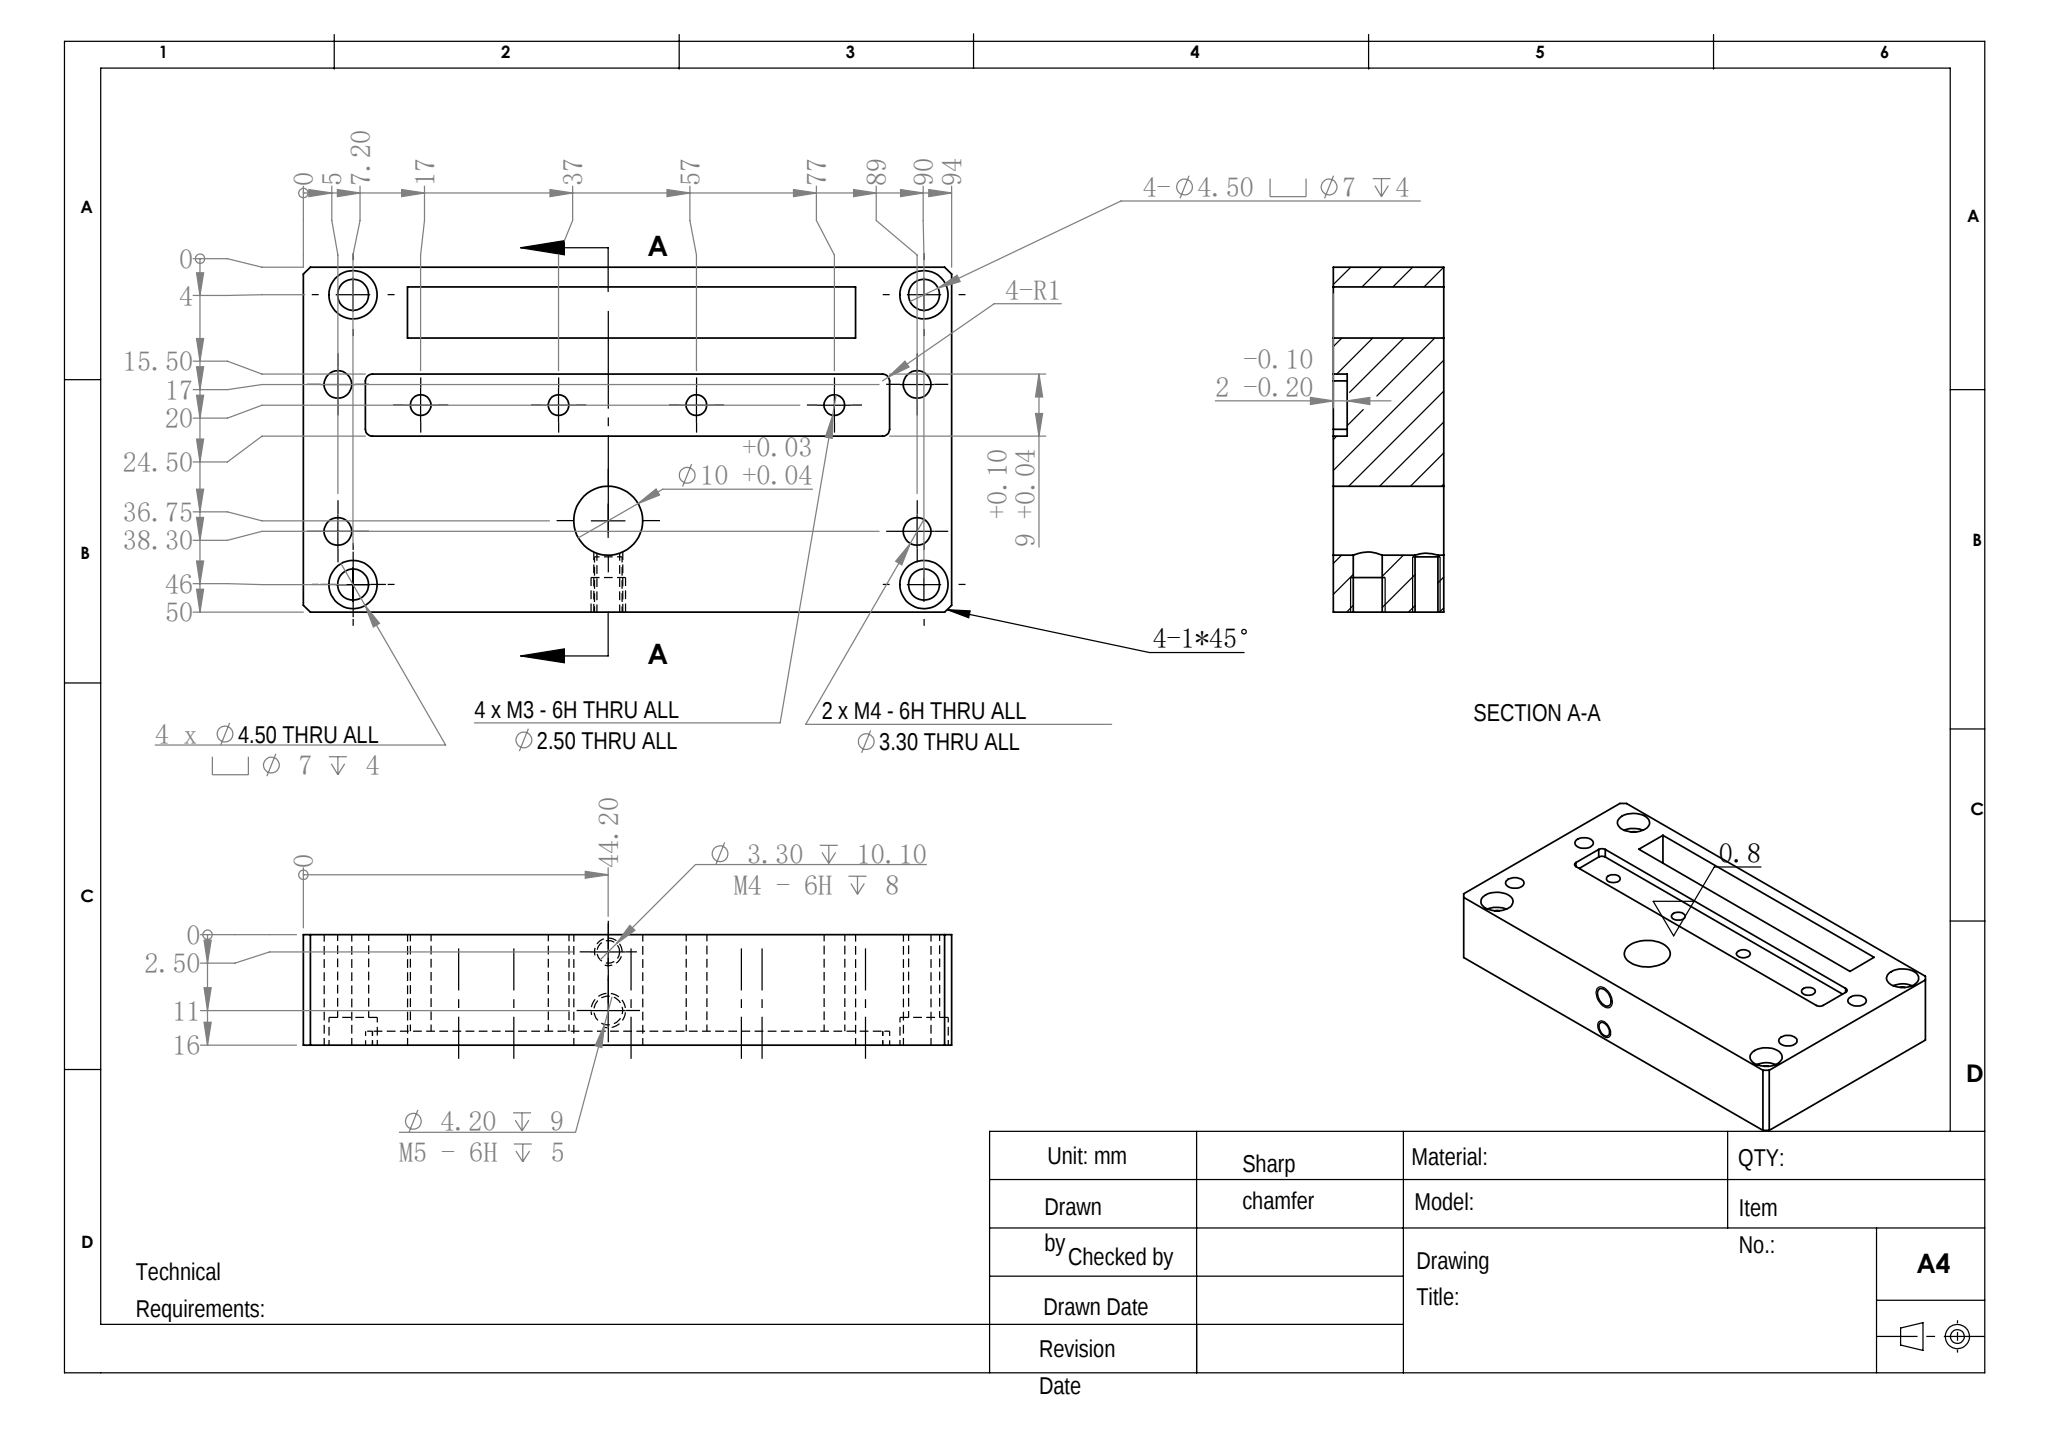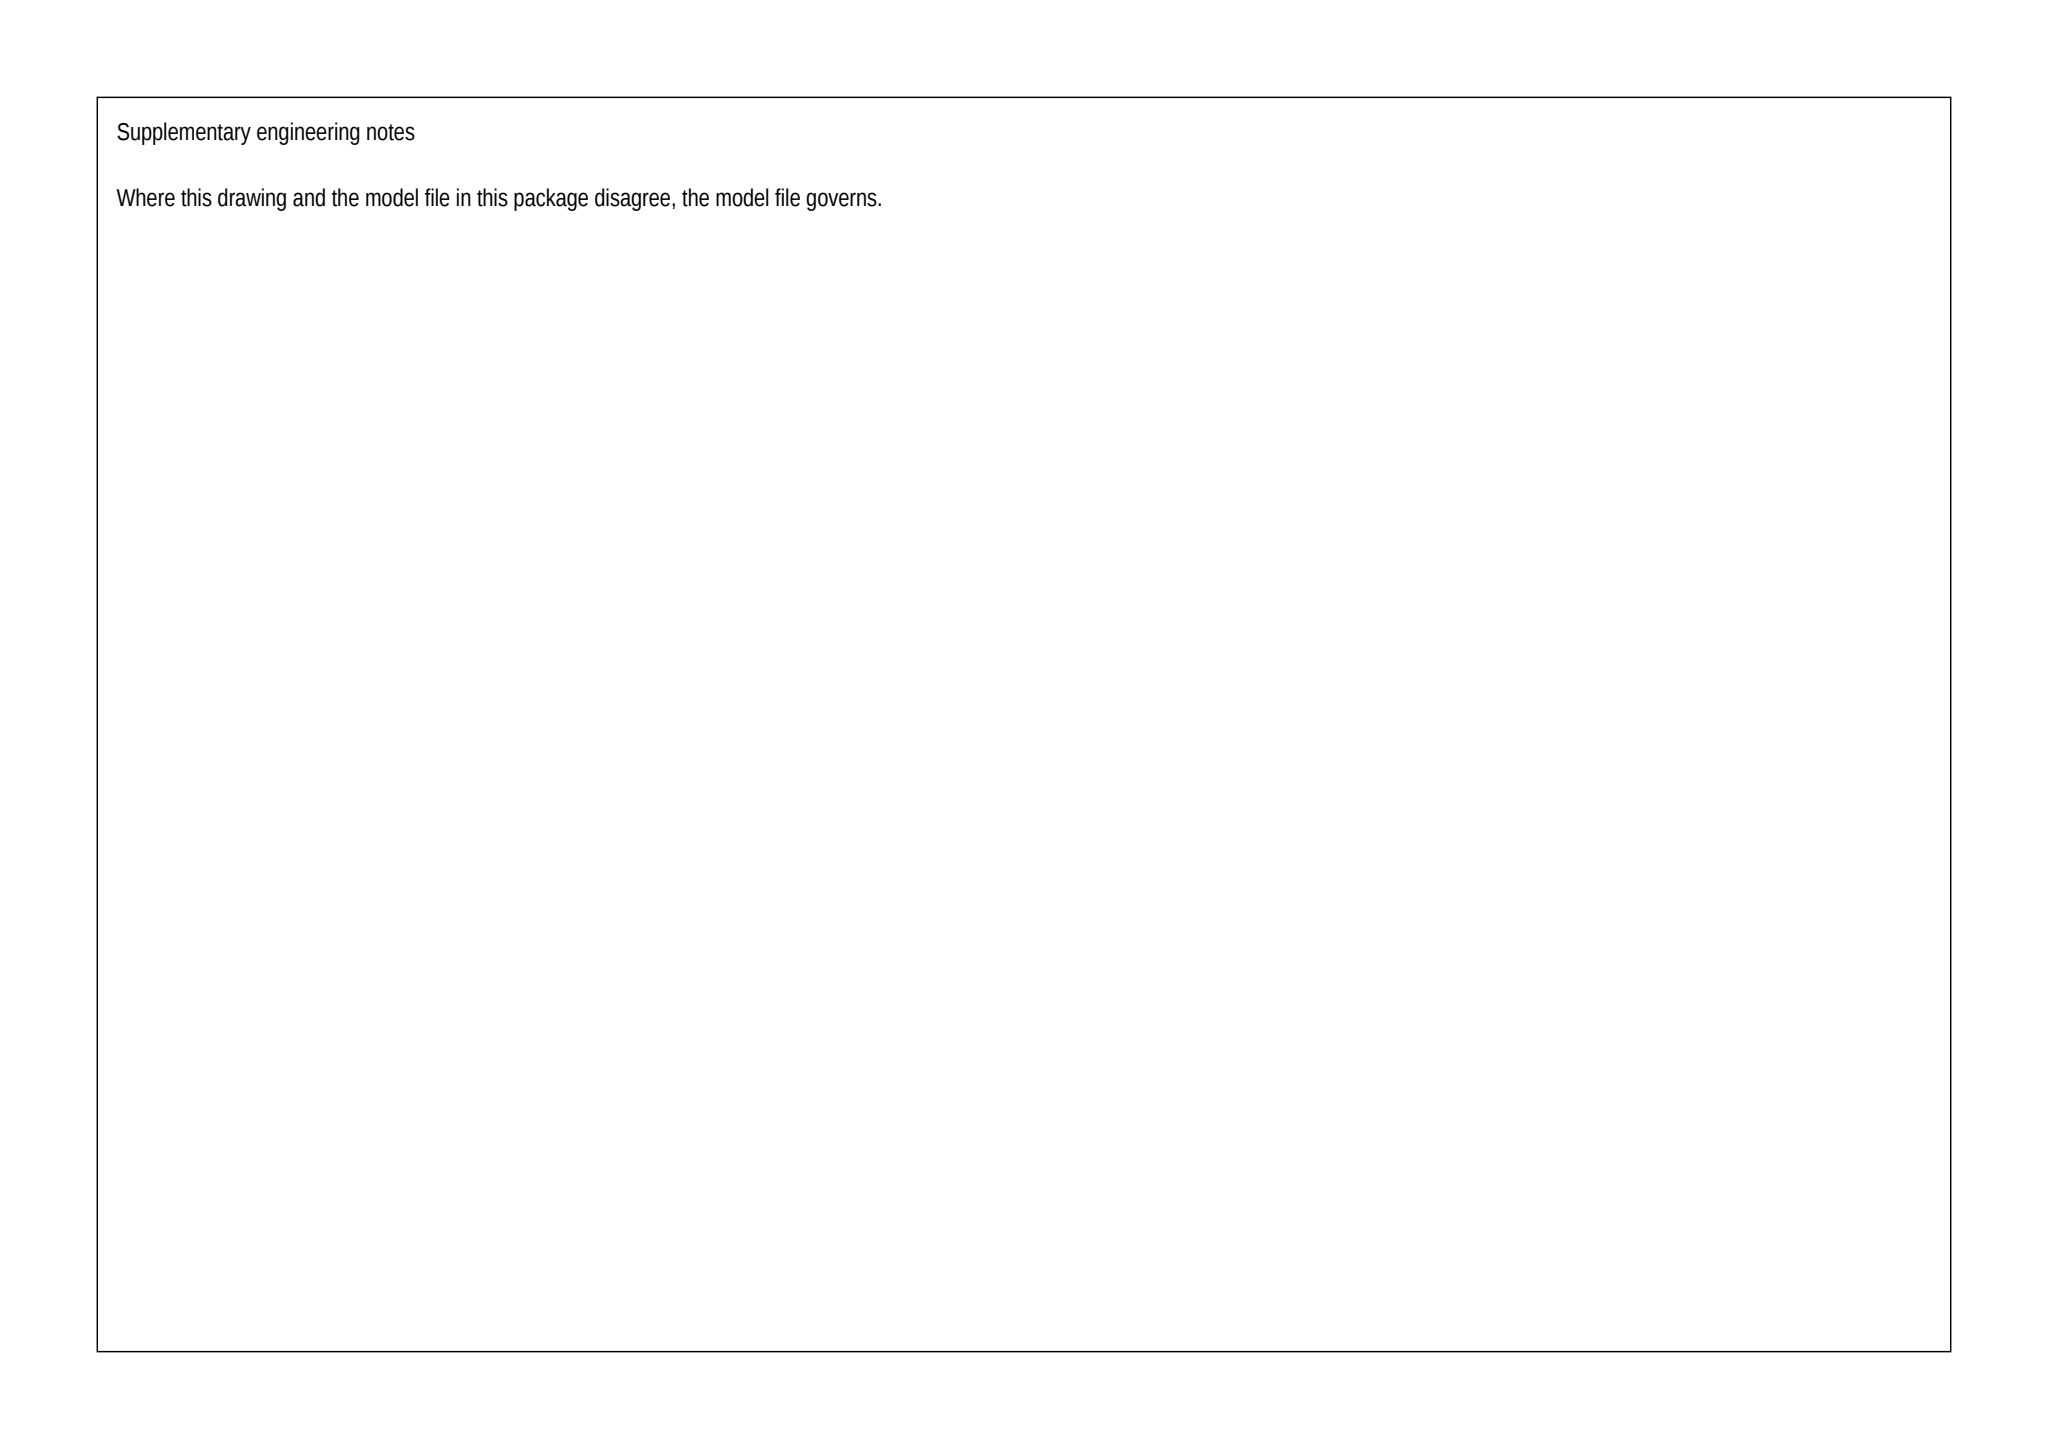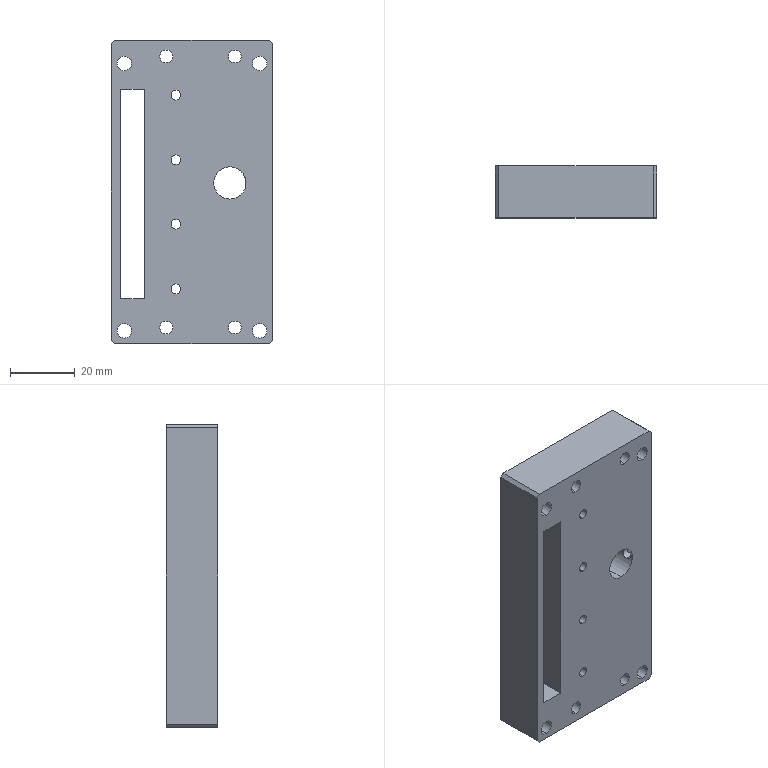Part | SolidWorks | mm | 1 solid | 65 faces | box 50 x 16 x 94 mm | volume 62074 mm3 | cylinder 42 | plane 23 | commonest cylinder face diameters 4 x8 3 x8 7 x8 4.5 x8 2 x4 3.3 x2 4.2 x2 10 x2
Drawing notes:
OVERALL 94 LG x 50 W x 16 THK | from the solid: bbox_xyz [50.0, 16.0, 94.0]
UPPER POCKET 64.97 LG x 7.41 W x 2 DP; 13.94 & 2.86 FROM 0 DATUMS | from the solid: z planes 13.94/78.91 (64.97 lg), x planes 2.86/10.27 (7.41 w), y 14.0 vs top 16.0 = 2 DP
Ø10 BORE CL 49.80 FROM LH EDGE (0 DATUM) | from the solid: cyl dia 10, axis y, pos_other_axes [36.75, null, 49.8], length 16 THRU
9 WIDE SLOT: 76 LG, FROM 9 TO 85 FROM LH EDGE | from the solid: z planes 9.0 and 85.0 bound slot between x planes 15.5/24.5 (9 wide)
9 WIDE SLOT FLOOR DP 4 FROM TOP FACE (12 ABOVE BOTTOM) | from the solid: y plane 12.0 slot floor, top face y=16, bbox y=16
4 X Ø4.50 CBORE Ø7 DP 4 AT 4 & 86.80 FROM LH EDGE | from the solid: Ø4.5/Ø7 cyls at z=4.0 and z=86.8, x=4.0 and 46.0
4 X M4-6H THRU ALL AT 5 & 89 FROM LH EDGE (WAS 2 X) | from the solid: four Ø4.0 y-axis thru holes at (x17,z5),(x17,z89),(x38.3,z5),(x38.3,z89), L=16
Ø10 +0.04/+0.03 THRU ALL (16 THK) | from the solid: cylinder dia 10.0, axis y, length 16.0 = full 16 mm part thickness
build123d program:
from build123d import *

# Parameters (mm, degrees)
BOSS_EXTRUDE1_DEPTH                             = 94
M4_HEX_SOCKET_HEAD_CAP_SCREW_CBORE1_D           = 4.5
M4_HEX_SOCKET_HEAD_CAP_SCREW_CBORE1_CBORE_D     = 7
M4_HEX_SOCKET_HEAD_CAP_SCREW_CBORE1_CBORE_DEPTH = 4
SKETCH4_R                                       = 5
CUT_EXTRUDE1_DEPTH                              = 30
M10_TAPPED_HOLE1_D                              = 10
M10_TAPPED_HOLE1_DEPTH                          = 6
M10_TAPPED_HOLE1_TIP                            = 3.004
M5_TAPPED_HOLE1_D                               = 4.2
M5_TAPPED_HOLE1_DEPTH                           = 9
M5_TAPPED_HOLE1_TIP                             = 1.262
BOSS_EXTRUDE2_START                             = 2
SKETCH19_W                                      = 18
SKETCH19_H                                      = 94
SKETCH19_R                                      = 5
BOSS_EXTRUDE2_DEPTH                             = 2
SKETCH20_W                                      = 9
SKETCH20_H                                      = 76
CUT_EXTRUDE3_DEPTH                              = 2
CHAMFER2_SIZE                                   = 1
M3_TAPPED_HOLE3_D                               = 3
FILLET1_R                                       = 1
M4_TAPPED_HOLE1_D                               = 3.3
M4_TAPPED_HOLE1_DEPTH                           = 10.1
M4_TAPPED_HOLE1_TIP                             = 0.9914
M4_TAPPED_HOLE2_D                               = 4
M4_TAPPED_HOLE3_D                               = 4
SKETCH37_W                                      = 7.412
SKETCH37_H                                      = 64.973
CUT_EXTRUDE4_DEPTH                              = 52


with BuildPart() as part:
    # Sketch1 → Boss-Extrude1 (new body)
    with BuildSketch(Plane.XY):
        Polygon((0, 0), (0, 16), (24, 16), (24, 14), (42, 14), (42, 16), (50, 16), (50, 0), align=None)
    extrude(amount=BOSS_EXTRUDE1_DEPTH)

    # M4 Hex Socket Head Cap Screw CBORE1 (through all)
    with Locations(Plane(origin=(0, 16, 0), x_dir=(-1, 0, 0), z_dir=(0, 1, 0))):
        with Locations((-46, 86.8), (-4, 86.8), (-4, 4), (-46, 4)):
            CounterBoreHole(M4_HEX_SOCKET_HEAD_CAP_SCREW_CBORE1_D / 2, M4_HEX_SOCKET_HEAD_CAP_SCREW_CBORE1_CBORE_D / 2, M4_HEX_SOCKET_HEAD_CAP_SCREW_CBORE1_CBORE_DEPTH)

    # Sketch4 → Cut-Extrude1 (cut)
    with BuildSketch(Plane(origin=(0, 16, 0), x_dir=(1, 0, 0), z_dir=(0, 1, 0))):
        with Locations(Location((36.75, -49.8, 0), (0, 0, 180))):
            Circle(SKETCH4_R)
    extrude(amount=-CUT_EXTRUDE1_DEPTH, mode=Mode.SUBTRACT)

    # M10 Tapped Hole1
    with Locations(Plane.XZ):
        with Locations((36.75, 49.8)):
            Hole(M10_TAPPED_HOLE1_D / 2, depth=M10_TAPPED_HOLE1_DEPTH)
            with Locations((0, 0, -(M10_TAPPED_HOLE1_DEPTH + M10_TAPPED_HOLE1_TIP / 2))):  # 118° drill point
                Cone(0, M10_TAPPED_HOLE1_D / 2, M10_TAPPED_HOLE1_TIP, mode=Mode.SUBTRACT)

    # M5 Tapped Hole1
    with Locations(Plane(origin=(50, -3.814, 7.875), x_dir=(0, 0, 1), z_dir=(1, 0, 0))):
        with Locations((41.925, -14.814)):
            Hole(M5_TAPPED_HOLE1_D / 2, depth=M5_TAPPED_HOLE1_DEPTH)
            with Locations((0, 0, -(M5_TAPPED_HOLE1_DEPTH + M5_TAPPED_HOLE1_TIP / 2))):  # 118° drill point
                Cone(0, M5_TAPPED_HOLE1_D / 2, M5_TAPPED_HOLE1_TIP, mode=Mode.SUBTRACT)

    # Sketch19 → Boss-Extrude2 (add)
    with BuildSketch(Plane(origin=(0, 14, 0), x_dir=(1, 0, 0), z_dir=(0, 1, 0)).offset(BOSS_EXTRUDE2_START)):
        with Locations((33, -47)):
            Rectangle(SKETCH19_W, SKETCH19_H)
        with Locations(Location((36.75, -49.8, 0), (0, 0, 180))):
            Circle(SKETCH19_R, mode=Mode.SUBTRACT)
    extrude(amount=-BOSS_EXTRUDE2_DEPTH)

    # Sketch20 → Cut-Extrude3 (cut)
    with BuildSketch(Plane(origin=(0, 16, 0), x_dir=(1, 0, 0), z_dir=(0, 1, 0))):
        with Locations((20, -47)):
            Rectangle(SKETCH20_W, SKETCH20_H)
    extrude(amount=-CUT_EXTRUDE3_DEPTH, mode=Mode.SUBTRACT)

    # Chamfer2
    chamfer2_edges = [part.edges().sort_by_distance(p)[0] for p in [
        (50, 8, 0),
        (0, 8, 94),
        (50, 8, 94),
        (0, 8, 0),
    ]]
    chamfer(chamfer2_edges, length=CHAMFER2_SIZE)

    # M3 Tapped Hole3 (through all)
    with Locations(Plane(origin=(0, 14, 0), x_dir=(1, 0, 0), z_dir=(0, 1, 0))):
        with Locations((20, -37), (20, -17), (20, -77), (20, -57)):
            Hole(M3_TAPPED_HOLE3_D / 2)

    # Fillet1
    fillet1_edges = [part.edges().sort_by_distance(p)[0] for p in [
        (15.5, 15, 85),
        (15.5, 15, 9),
        (24.5, 15, 9),
        (24.5, 15, 85),
    ]]
    fillet(fillet1_edges, radius=FILLET1_R)

    # M4 Tapped Hole1
    with Locations(Plane(origin=(50, 0, 0), x_dir=(0, 0, -1), z_dir=(1, 0, 0))):
        with Locations((-49.8, 2.5)):
            Hole(M4_TAPPED_HOLE1_D / 2, depth=M4_TAPPED_HOLE1_DEPTH)
            with Locations((0, 0, -(M4_TAPPED_HOLE1_DEPTH + M4_TAPPED_HOLE1_TIP / 2))):  # 118° drill point
                Cone(0, M4_TAPPED_HOLE1_D / 2, M4_TAPPED_HOLE1_TIP, mode=Mode.SUBTRACT)

    # M4 Tapped Hole2 (through all)
    with Locations(Plane(origin=(0, 16, 0), x_dir=(1, 0, 0), z_dir=(0, 1, 0))):
        with Locations((38.3, -89), (17, -89)):
            Hole(M4_TAPPED_HOLE2_D / 2)

    # M4 Tapped Hole3 (through all)
    with Locations(Plane(origin=(0, 16, 0), x_dir=(1, 0, 0), z_dir=(0, 1, 0))):
        with Locations((38.3, -5), (17, -5)):
            Hole(M4_TAPPED_HOLE3_D / 2)

    # Sketch37 → Cut-Extrude4 (cut)
    with BuildSketch(Plane(origin=(0, 16, 0), x_dir=(1, 0, 0), z_dir=(0, 1, 0))):
        with Locations((6.567, -46.422)):
            Rectangle(SKETCH37_W, SKETCH37_H)
    extrude(amount=-CUT_EXTRUDE4_DEPTH, mode=Mode.SUBTRACT)


solid = part.part